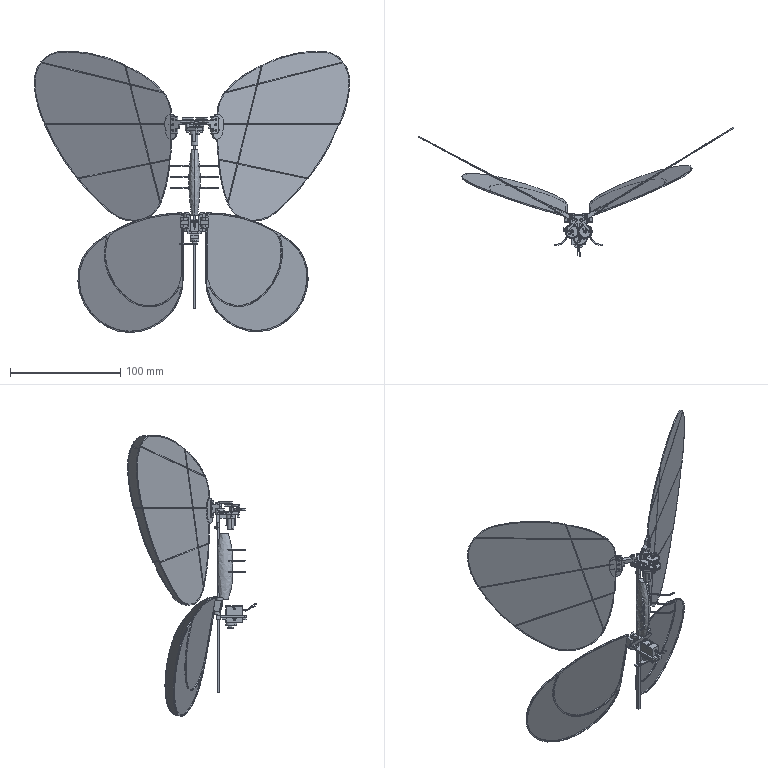Assembly | SolidWorks | mm | 18 component files | 20 solids | 3831 faces | box 286.46 x 116.99 x 255.2 mm | volume 18300 mm3 | cylinder 2904 | plane 551 | spline 338 | torus 31 | sphere 4 | cone 3 | commonest cylinder face diameters 0.228 x333 0.344 x221 0.811 x172 0.44 x172 0.528 x135 0.449 x133 11.25 x123 12.6 x120
Bill of materials:
AileronConnector10 | 1 |  | Symmetric H-shaped yoke or bracket body. It has four rounded lobes, each with a small hole, joined by curved webs, plus a long flat strip with rounded ends passing crosswise through the middle.
ConnectingRod | 2 |  | Flat link or arm of constant thickness. Both ends are rounded, the waist is narrow and slightly curved, and there is a small hole at one end and a larger hole at the other.
ConnectingRodGearStraightToothM0.3X40 | 2 |  | Flat spur-gear-like disc with straight external teeth around the rim (roughly 40, not counted exactly). It has an off-center hollow cylindrical boss that sticks out on both faces, plus a second, shorter off-center cylindrical boss on the underside at a different position. The web has several round through-holes of different sizes and shallow grooves on the top face.
CorelessMotor | 1 |  | Plain cylindrical body with a slightly rounded top edge. A short, wider collar on the top face carries a thin coaxial pin or shaft.
FrontWing1-G2 | 1 |  | Very thin, flat, rounded-teardrop panel. A small rounded tab with three small holes sits on one edge, and faint lines across the surface divide it into segments.
FrontWing2 | 1 |  | Very thin, flat, rounded-teardrop panel. A small tab with three small holes sits on one edge, and straight lines across the face divide it into segments. It appears to be the mirror image of the similar panel.
MotorDriveGearStraightToothM0.3X7 | 1 |  | Small, tall pinion-like cylinder with about 8 rounded, straight external teeth running the full length of the body. It has a central through-bore and a thin round flange at one end.
RearWing1-G | 1 |  | Thin, slightly curved or dished teardrop-shaped shell or plate. One straight edge carries a small bracket or tab with a small hole, and an inner curved line or step sits concentric with the outer edge.
RearWing2-G | 1 |  | Thin teardrop-shaped plate or shell. A small tab with a hole sits at one end of the straight edge, and an inner curved rim line runs parallel to the outer edge.
ReductionGearStraightToothM0.3X40 | 1 |  | Compound gear-like part: a large, thin disc with straight external teeth (roughly 40) plus a small coaxial toothed pinion (about 10 teeth) rising from one face. A plain cylindrical hub sticks out from the opposite face. There is a small central bore, and three large round through-holes are spaced around the center of the web.
ServoHanger | 1 |  | Flat rectangular frame plate with a large rectangular central cutout and narrower tabs at both ends. Each tab has a round hole, and one tab also has a square hole. One end has a stepped, thicker region.
sg90 | 1 |  | Rectangular box-shaped body with a mounting flange on both sides, each with a slotted hole. A stepped cylindrical boss on one face carries a tapered arm with three small holes, and two flexible wire-like strands exit one end.
SquareRod | 1 |  | Long thin straight rod with an elongated spindle- or oval-shaped body attached along one side near one end. Three pairs of thin, curved, wire-like legs project from the body on opposite sides.
SwingRod | 2 |  | Bracket with a flat plate that has three through-holes, a rounded corner, and an open slot or fork at its top. An offset arm leads to two adjacent hollow cylindrical bosses of different heights.
WingDriveSupport | 1 |  | Complex plate-type housing or mount. It has a tapered outline, a large central round opening ringed by a circular boss with radiating ribs, small corner holes, raised cylindrical bosses, downward legs or standoffs, and a small knob or pin on one edge.
Mates:
1. concentric | WingDriveSupport-1 face at (0.5486, -2.426, 21.25) dir (0, 0, 1) r 3.5 | CorelessMotor-1 face at (0.5486, -2.426, 26.25) dir (0, 0, -1) r 3
2. coincident | WingDriveSupport-1 face at (0.5486, -2.426, 26.25) dir (0, 0, -1) | CorelessMotor-1 face at (0.5486, -2.426, 26.25) dir (0, 0, 1)
3. concentric | CorelessMotor-1 face at (0.5486, -2.426, 30.97) dir (0, 0, -1) r 0.5 | MotorDriveGearStraightToothM0.3X7-1 face at (0.5486, -2.426, 30.32) dir (0, 0, -1) r 1.35
4. coincident | CorelessMotor-1 face at (0.5486, -2.426, 26.65) dir (0, 0, 1) | MotorDriveGearStraightToothM0.3X7-1 face at (0.5486, -2.426, 26.65) dir (0, 0, -1)
5. concentric | WingDriveSupport-1 face at (2.303, -9.254, 24.75) dir (0, 0, 1) r 0.5 | ReductionGearStraightToothM0.3X40-1 face at (2.303, -9.254, 34.15) dir (0, 0, -1) r 0.5
6. coincident | WingDriveSupport-1 face at (0.5486, -3.254, 27.25) dir (0, 0, 1) | ReductionGearStraightToothM0.3X40-1 face at (2.303, -9.254, 27.25) dir (0, 0, -1)
7. concentric | WingDriveSupport-1 face at (-5.451, -3.254, 24.75) dir (0, 0, 1) r 0.5 | ConnectingRodGearStraightToothM0.3X40-2 face at (-5.451, -3.254, 42.15) dir (0, 0, -1) r 0.5
8. concentric | WingDriveSupport-1 face at (6.549, -3.254, 24.75) dir (0, 0, 1) r 0.5 | ConnectingRodGearStraightToothM0.3X40-3 face at (6.549, -3.254, 42.15) dir (0, 0, -1) r 0.5
9. gear | MotorDriveGearStraightToothM0.3X7-1 edge at (0.5486, -2.426, 30.32) dir (0, 0, 1) r 0.5 | ReductionGearStraightToothM0.3X40-1 edge at (2.303, -9.254, 33.5) dir (0, 0, 1) r 0.5
10. gear | ReductionGearStraightToothM0.3X40-1 face at (2.303, -9.254, 34.15) dir (0, 0, -1) r 0.5 | ConnectingRodGearStraightToothM0.3X40-3 face at (6.549, -3.254, 42.15) dir (0, 0, -1) r 0.5
11. concentric | ConnectingRodGearStraightToothM0.3X40-2 face at (-9.354, -2.379, 34.75) dir (0, 0, -1) r 0.5 | ConnectingRod-3 face at (-9.354, -2.379, 37.25) dir (0, 0, -1) r 0.5
12. concentric | ConnectingRodGearStraightToothM0.3X40-3 face at (10.508, -2.687, 34.75) dir (0, 0, -1) r 0.5 | ConnectingRod-4 face at (10.508, -2.687, 37.25) dir (0, 0, -1) r 0.5
13. concentric | WingDriveSupport-1 face at (-6.202, 9.324, 29.75) dir (0, 0, -1) r 1 | SwingRod-1 face at (-6.202, 9.324, 29.099) dir (0, 0, 1) r 1
14. coincident | WingDriveSupport-1 face at (0.5486, -3.254, 29.75) dir (0, 0, 1) | SwingRod-1 face at (-1.962, 7.074, 29.75) dir (0, 0, -1)
15. concentric | ConnectingRod-3 face at (-1.962, 7.074, 37.25) dir (0, 0, -1) r 1 | SwingRod-1 face at (-1.962, 7.074, 29.099) dir (0, 0, 1) r 1
16. concentric | WingDriveSupport-1 face at (7.299, 9.324, 29.75) dir (0, 0, -1) r 1 | SwingRod-2 face at (7.299, 9.324, 29.099) dir (0, 0, 1) r 1
17. coincident | WingDriveSupport-1 face at (0.5486, -3.254, 29.75) dir (0, 0, 1) | SwingRod-2 face at (3.199, 6.829, 29.75) dir (0, 0, -1)
18. concentric | ConnectingRod-4 face at (3.199, 6.829, 37.25) dir (0, 0, -1) r 1 | SwingRod-2 face at (3.199, 6.829, 29.099) dir (0, 0, 1) r 1
19. coincident | ConnectingRod-4 face at (10.508, -2.687, 34.75) dir (0, 0, -1) | SwingRod-2 face at (3.199, 6.829, 34.75) dir (0, 0, 1)
20. coincident | ConnectingRod-3 face at (-9.354, -2.379, 34.75) dir (0, 0, -1) | SwingRod-1 face at (-1.962, 7.074, 34.75) dir (0, 0, 1)
21. gear | ConnectingRodGearStraightToothM0.3X40-2 face at (-5.451, -3.254, 42.15) dir (0, 0, -1) r 0.5 | ConnectingRodGearStraightToothM0.3X40-3 face at (6.549, -3.254, 42.15) dir (0, 0, -1) r 0.5
22. coincident | WingDriveSupport-1 face at (-0.4514, 9.746, 17.75) dir (0, -1, 0) | SquareRod-1 face at (1.549, 9.746, 22.75) dir (0, 1, 0)
23. coincident | WingDriveSupport-1 face at (1.549, 9.746, 17.75) dir (-1, 0, 0) | SquareRod-1 face at (1.549, 7.746, 22.75) dir (1, 0, 0)
24. coincident | WingDriveSupport-1 face at (0.5486, -3.254, 17.75) dir (0, 0, -1) | SquareRod-1 face at (-8.451, 14.606, 17.75) dir (0, 0, 1)
25. width | AileronConnector10-1 face at (-0.5014, 8.796, -58.554) dir (1, 0, 0) | AileronConnector10-1 face at (1.599, 8.796, -58.554) dir (-1, 0, 0) | SquareRod-1 face at (-0.4514, 7.746, 22.75) dir (-1, 0, 0) | SquareRod-1 face at (1.549, 7.746, 22.75) dir (1, 0, 0)
26. coincident | SquareRod-1 face at (1.549, 7.746, 22.75) dir (0, -1, 0) | AileronConnector10-1 face at (1.599, 7.746, -56.708) dir (0, 1, 0)
27. coincident | SquareRod-1 face at (-0.4514, 7.746, 22.75) dir (-1, 0, 0) | ServoHanger-1 face at (-0.4514, 7.746, -67.03) dir (1, 0, 0)
28. coincident | SquareRod-1 face at (1.549, 7.746, 22.75) dir (0, -1, 0) | ServoHanger-1 face at (-0.4514, 7.746, -67.03) dir (0, 1, 0)
29. coincident | ServoHanger-1 face at (0.5986, 8.796, -69.03) dir (0, 0, -1) | sg90-1 face at (0.5986, -5.577, -69.03) dir (0, 0, 1)
30. coincident | ServoHanger-1 face at (-3.401, -13.204, -67.03) dir (1, 0, 0) | sg90-1 face at (-3.401, -5.577, -70.725) dir (-1, 0, 0)
31. coincident | ServoHanger-1 face at (4.599, -13.204, -67.03) dir (0, 1, 0) | sg90-1 face at (-3.401, -13.204, -73.64) dir (0, -1, 0)
32. distance | ServoHanger-1 face at (0.5986, 8.796, -67.03) dir (0, 0, 1) | CorelessMotor-1 face at (0.5486, -2.426, 10.97) dir (0, 0, -1)
33. tangent | AileronConnector10-1 face at (-5.451, 6.884, -64.984) dir (0, 0.9848, 0.1736) r 2 | ServoHanger-1 edge at (-2.401, 6.796, -67.03) dir (-1, 0, 0)
34. concentric | AileronConnector10-1 face at (8.849, 7.407, -50.675) dir (0, 0.1736, -0.9848) r 0.5 | RearWing2-G-1 face at (8.849, 27.358, -163.826) dir (0, -0.1736, 0.9848) r 0.5
35. width | AileronConnector10-1 face at (7.549, -5.306, -55.839) dir (0, 0.1736, -0.9848) | AileronConnector10-1 face at (0.5486, 9.682, -63.576) dir (0, -0.1736, 0.9848) | RearWing2-G-1 face at (13.623, 6.464, -53.876) dir (0, -0.1736, 0.9848) | RearWing2-G-1 face at (13.623, 8.201, -63.724) dir (0, 0.1736, -0.9848)
36. concentric | AileronConnector10-1 face at (-7.751, 7.407, -50.675) dir (0, 0.1736, -0.9848) r 0.5 | RearWing1-G-1 face at (-7.751, 27.358, -163.826) dir (0, -0.1736, 0.9848) r 0.5
37. width | AileronConnector10-1 face at (-6.451, -5.306, -55.839) dir (0, 0.1736, -0.9848) | AileronConnector10-1 face at (0.5486, 9.682, -63.576) dir (0, -0.1736, 0.9848) | RearWing1-G-1 face at (-12.385, 6.075, -53.945) dir (0, -0.1736, 0.9848) | RearWing1-G-1 face at (-12.385, 7.811, -63.793) dir (0, 0.1736, -0.9848)
38. concentric | SwingRod-2 face at (18.068, 17.983, 34.75) dir (0.5198, -0.8543, 0) r 1 | FrontWing1-G2-1 face at (19.523, 15.591, 34.75) dir (-0.5198, 0.8543, 0) r 1
39. concentric | SwingRod-2 face at (18.068, 17.983, 29.75) dir (0.5198, -0.8543, 0) r 1 | FrontWing1-G2-1 face at (19.523, 15.591, 29.75) dir (-0.5198, 0.8543, 0) r 1
40. coincident | SwingRod-2 face at (16.348, 16, 37.934) dir (0.5198, -0.8543, 0) | FrontWing1-G2-1 face at (20.718, 18.658, 34.362) dir (-0.5198, 0.8543, 0)
41. coincident | WingDriveSupport-1 face at (6.549, -3.254, 31.25) dir (0, 0, 1) | ConnectingRodGearStraightToothM0.3X40-3 face at (6.549, -3.254, 31.25) dir (0, 0, -1)
42. coincident | WingDriveSupport-1 face at (-5.451, -3.254, 31.25) dir (0, 0, 1) | ConnectingRodGearStraightToothM0.3X40-2 face at (-5.451, -3.254, 31.25) dir (0, 0, -1)
43. coincident | SwingRod-1 face at (-16.564, 13.691, 37.934) dir (0.4688, 0.8833, 0) | FrontWing2-1 face at (-21.082, 16.089, 34.362) dir (-0.4688, -0.8833, 0)
44. concentric | SwingRod-1 edge at (-17.483, 17.292, 29.75) dir (0.4688, 0.8833, 0) r 1 | FrontWing2-1 edge at (-17.835, 16.629, 29.75) dir (0.4688, 0.8833, 0) r 1
45. concentric | SwingRod-1 face at (-19.147, 14.156, 24.75) dir (0.4688, 0.8833, 0) r 1 | FrontWing2-1 face at (-18.772, 14.863, 24.75) dir (0.4688, 0.8833, 0) r 1